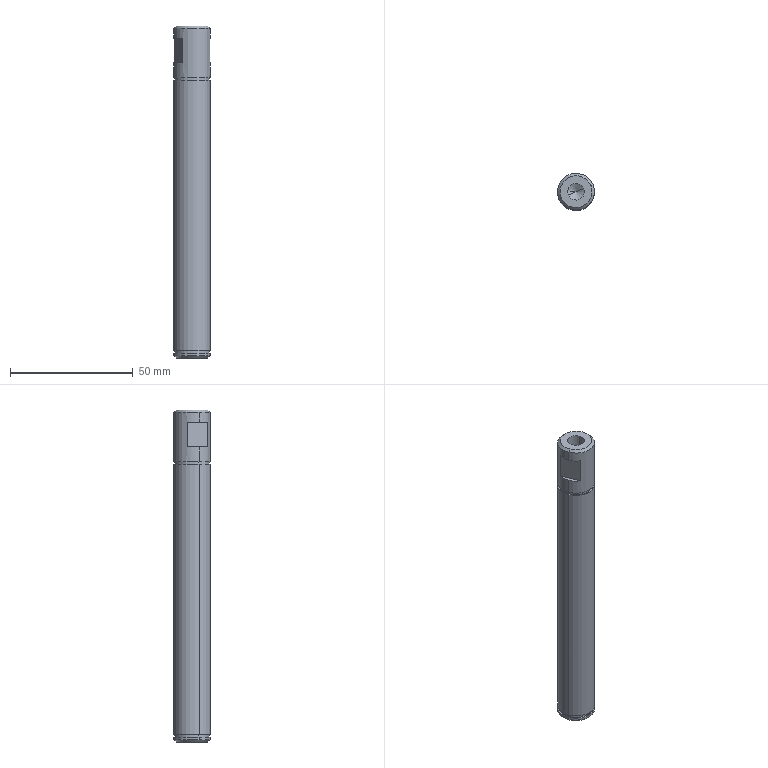Component | SolidWorks | TAR-01-28PaperSupportRollerAxis-1 | 1 solid | 30 faces | box 15 x 15 x 135.2 mm | volume 22680 mm3 | cylinder 12 | plane 12 | cone 6 | commonest cylinder face diameters 15 x6 14 x4 6.8 x2
build123d program:
from build123d import *

# Parameters (mm, degrees)
SKETCH1_R             = 7.5
BOSS_EXTRUDE1_DEPTH   = 5
BOSS_EXTRUDE2_DEPTH   = 10
SKETCH3_R             = 7.5
BOSS_EXTRUDE3_DEPTH   = 6
SKETCH4_R             = 7
BOSS_EXTRUDE4_DEPTH   = 1.1
SKETCH5_R             = 7.5
BOSS_EXTRUDE5_DEPTH   = 110
SKETCH6_R             = 7
BOSS_EXTRUDE6_DEPTH   = 1.1
SKETCH7_R             = 7.5
BOSS_EXTRUDE7_DEPTH   = 2
CHAMFER1_SIZE         = 1
M8_TAPPED_HOLE2_D     = 6.8
M8_TAPPED_HOLE2_DEPTH = 25
M8_TAPPED_HOLE2_TIP   = 2.043


with BuildPart() as part:
    # Sketch1 → Boss-Extrude1 (new body)
    with BuildSketch(Plane.XY):
        Circle(SKETCH1_R)
    extrude(amount=BOSS_EXTRUDE1_DEPTH)

    # Sketch2 → Boss-Extrude2 (add)
    with BuildSketch(Plane.XY.offset(5)):
        with BuildLine():
            Line((6, -4.5), (6, 4.5))
            ThreePointArc((6, 4.5), (0, 7.5), (-6, 4.5))
            Line((-6, 4.5), (-6, -4.5))
            ThreePointArc((-6, -4.5), (0, -7.5), (6, -4.5))
        make_face()
    extrude(amount=BOSS_EXTRUDE2_DEPTH)

    # Sketch3 → Boss-Extrude3 (add)
    with BuildSketch(Plane.XY.offset(15)):
        Circle(SKETCH3_R)
    extrude(amount=BOSS_EXTRUDE3_DEPTH)

    # Sketch4 → Boss-Extrude4 (add)
    with BuildSketch(Plane.XY.offset(21)):
        Circle(SKETCH4_R)
    extrude(amount=BOSS_EXTRUDE4_DEPTH)

    # Sketch5 → Boss-Extrude5 (add)
    with BuildSketch(Plane.XY.offset(22.1)):
        Circle(SKETCH5_R)
    extrude(amount=BOSS_EXTRUDE5_DEPTH)

    # Sketch6 → Boss-Extrude6 (add)
    with BuildSketch(Plane.XY.offset(132.1)):
        Circle(SKETCH6_R)
    extrude(amount=BOSS_EXTRUDE6_DEPTH)

    # Sketch7 → Boss-Extrude7 (add)
    with BuildSketch(Plane.XY.offset(133.2)):
        Circle(SKETCH7_R)
    extrude(amount=BOSS_EXTRUDE7_DEPTH)

    # Chamfer1
    chamfer1_edges = [part.edges().sort_by_distance(p)[0] for p in [
        (-7.5, 0, 0),
        (-7.5, 0, 135.2),
    ]]
    chamfer(chamfer1_edges, length=CHAMFER1_SIZE)

    # M8 Tapped Hole2
    with Locations(Plane(origin=(0, 0, 0), x_dir=(-1, 0, 0), z_dir=(0, 0, -1))):
        with Locations((0, 0)):
            Hole(M8_TAPPED_HOLE2_D / 2, depth=M8_TAPPED_HOLE2_DEPTH)
            with Locations((0, 0, -(M8_TAPPED_HOLE2_DEPTH + M8_TAPPED_HOLE2_TIP / 2))):  # 118° drill point
                Cone(0, M8_TAPPED_HOLE2_D / 2, M8_TAPPED_HOLE2_TIP, mode=Mode.SUBTRACT)


solid = part.part

# Placed as in the assembly
solid = solid.moved(Location((100.319, 9.938, -9.5), (-180, 0, -22.523)))
STEP:
#1=CARTESIAN_POINT('',(3.826,0.34,-1.358));
#2=VERTEX_POINT('',#1);
#3=CARTESIAN_POINT('',(4.073,0.4425,-1.358));
#4=VERTEX_POINT('',#3);
#5=CARTESIAN_POINT('',(3.95,0.3912,-1.358));
#6=DIRECTION('',(0.,0.,1.));
#7=DIRECTION('',(0.9237,0.383,0.));
#8=AXIS2_PLACEMENT_3D('',#5,#6,#7);
#9=CIRCLE('',#8,0.1339);
#10=EDGE_CURVE('',#2,#4,#9,.T.);
#11=ORIENTED_EDGE('',*,*,#10,.F.);
#12=CARTESIAN_POINT('',(3.826,0.34,-0.374));
#13=VERTEX_POINT('',#12);
#14=CARTESIAN_POINT('',(3.826,0.34,-0.374));
#15=DIRECTION('',(0.,0.,1.));
#16=VECTOR('',#15,39.37);
#17=LINE('',#14,#16);
#18=EDGE_CURVE('',#2,#13,#17,.T.);
#19=ORIENTED_EDGE('',*,*,#18,.T.);
#20=CARTESIAN_POINT('',(4.073,0.4425,-0.374));
#21=VERTEX_POINT('',#20);
#22=CARTESIAN_POINT('',(3.95,0.3912,-0.374));
#23=DIRECTION('',(0.,0.,1.));
#24=DIRECTION('',(0.9237,0.383,0.));
#25=AXIS2_PLACEMENT_3D('',#22,#23,#24);
#26=CIRCLE('',#25,0.1339);
#27=EDGE_CURVE('',#13,#21,#26,.T.);
#28=ORIENTED_EDGE('',*,*,#27,.T.);
#29=CARTESIAN_POINT('',(4.073,0.4425,-0.374));
#30=DIRECTION('',(0.,0.,1.));
#31=VECTOR('',#30,39.37);
#32=LINE('',#29,#31);
#33=EDGE_CURVE('',#4,#21,#32,.T.);
#34=ORIENTED_EDGE('',*,*,#33,.F.);
#35=EDGE_LOOP('',(#11,#19,#28,#34));
#36=FACE_OUTER_BOUND('',#35,.T.);
#37=CARTESIAN_POINT('',(3.95,0.3912,-0.374));
#38=DIRECTION('',(0.,0.,1.));
#39=DIRECTION('',(0.9237,0.383,0.));
#40=AXIS2_PLACEMENT_3D('',#37,#38,#39);
#41=CYLINDRICAL_SURFACE('',#40,0.1339);
#42=ADVANCED_FACE('',(#36),#41,.F.);
#43=CARTESIAN_POINT('',(3.95,0.3912,-1.439));
#44=VERTEX_POINT('',#43);
#45=CARTESIAN_POINT('',(4.073,0.4425,-1.358));
#46=DIRECTION('',(0.7918,0.3283,0.515));
#47=VECTOR('',#46,39.37);
#48=LINE('',#45,#47);
#49=EDGE_CURVE('',#44,#4,#48,.T.);
#50=ORIENTED_EDGE('',*,*,#49,.F.);
#51=CARTESIAN_POINT('',(3.826,0.34,-1.358));
#52=DIRECTION('',(-0.7918,-0.3283,0.515));
#53=VECTOR('',#52,39.37);
#54=LINE('',#51,#53);
#55=EDGE_CURVE('',#44,#2,#54,.T.);
#56=ORIENTED_EDGE('',*,*,#55,.T.);
#57=ORIENTED_EDGE('',*,*,#10,.T.);
#58=EDGE_LOOP('',(#50,#56,#57));
#59=FACE_OUTER_BOUND('',#58,.T.);
#60=CARTESIAN_POINT('',(3.95,0.3912,-1.358));
#61=DIRECTION('',(0.,0.,1.));
#62=DIRECTION('',(0.9237,0.383,0.));
#63=AXIS2_PLACEMENT_3D('',#60,#61,#62);
#64=CONICAL_SURFACE('',#63,0.1339,1.03);
#65=ADVANCED_FACE('',(#59),#64,.F.);
#66=CARTESIAN_POINT('',(3.713,0.2932,-5.697));
#67=VERTEX_POINT('',#66);
#68=CARTESIAN_POINT('',(4.186,0.4893,-5.697));
#69=VERTEX_POINT('',#68);
#70=CARTESIAN_POINT('',(3.95,0.3912,-5.697));
#71=DIRECTION('',(0.,0.,-1.));
#72=DIRECTION('',(-0.9237,-0.383,0.));
#73=AXIS2_PLACEMENT_3D('',#70,#71,#72);
#74=CIRCLE('',#73,0.2559);
#75=EDGE_CURVE('',#67,#69,#74,.T.);
#76=ORIENTED_EDGE('',*,*,#75,.F.);
#77=CARTESIAN_POINT('',(3.677,0.2781,-5.657));
#78=VERTEX_POINT('',#77);
#79=CARTESIAN_POINT('',(3.713,0.2932,-5.697));
#80=DIRECTION('',(-0.6532,-0.2709,0.7071));
#81=VECTOR('',#80,39.37);
#82=LINE('',#79,#81);
#83=EDGE_CURVE('',#67,#78,#82,.T.);
#84=ORIENTED_EDGE('',*,*,#83,.T.);
#85=CARTESIAN_POINT('',(4.222,0.5044,-5.657));
#86=VERTEX_POINT('',#85);
#87=CARTESIAN_POINT('',(3.95,0.3912,-5.657));
#88=DIRECTION('',(0.,0.,1.));
#89=DIRECTION('',(-0.9237,-0.383,0.));
#90=AXIS2_PLACEMENT_3D('',#87,#88,#89);
#91=CIRCLE('',#90,0.2953);
#92=EDGE_CURVE('',#86,#78,#91,.T.);
#93=ORIENTED_EDGE('',*,*,#92,.F.);
#94=CARTESIAN_POINT('',(4.186,0.4893,-5.697));
#95=DIRECTION('',(0.6532,0.2709,0.7071));
#96=VECTOR('',#95,39.37);
#97=LINE('',#94,#96);
#98=EDGE_CURVE('',#69,#86,#97,.T.);
#99=ORIENTED_EDGE('',*,*,#98,.F.);
#100=EDGE_LOOP('',(#76,#84,#93,#99));
#101=FACE_OUTER_BOUND('',#100,.T.);
#102=CARTESIAN_POINT('',(3.95,0.3912,-5.697));
#103=DIRECTION('',(0.,0.,1.));
#104=DIRECTION('',(0.9237,0.383,0.));
#105=AXIS2_PLACEMENT_3D('',#102,#103,#104);
#106=CONICAL_SURFACE('',#105,0.2559,0.7854);
#107=ADVANCED_FACE('',(#101),#106,.T.);
#108=CARTESIAN_POINT('',(4.186,0.4893,-0.374));
#109=VERTEX_POINT('',#108);
#110=CARTESIAN_POINT('',(3.713,0.2932,-0.374));
#111=VERTEX_POINT('',#110);
#112=CARTESIAN_POINT('',(3.95,0.3912,-0.374));
#113=DIRECTION('',(0.,0.,1.));
#114=DIRECTION('',(-0.9237,-0.383,0.));
#115=AXIS2_PLACEMENT_3D('',#112,#113,#114);
#116=CIRCLE('',#115,0.2559);
#117=EDGE_CURVE('',#109,#111,#116,.T.);
#118=ORIENTED_EDGE('',*,*,#117,.F.);
#119=CARTESIAN_POINT('',(4.222,0.5044,-0.4134));
#120=VERTEX_POINT('',#119);
#121=CARTESIAN_POINT('',(4.222,0.5044,-0.4134));
#122=DIRECTION('',(0.6532,0.2709,-0.7071));
#123=VECTOR('',#122,39.37);
#124=LINE('',#121,#123);
#125=EDGE_CURVE('',#109,#120,#124,.T.);
#126=ORIENTED_EDGE('',*,*,#125,.T.);
#127=CARTESIAN_POINT('',(3.677,0.2781,-0.4134));
#128=VERTEX_POINT('',#127);
#129=CARTESIAN_POINT('',(3.95,0.3912,-0.4134));
#130=DIRECTION('',(0.,0.,-1.));
#131=DIRECTION('',(-0.9237,-0.383,0.));
#132=AXIS2_PLACEMENT_3D('',#129,#130,#131);
#133=CIRCLE('',#132,0.2953);
#134=EDGE_CURVE('',#128,#120,#133,.T.);
#135=ORIENTED_EDGE('',*,*,#134,.F.);
#136=CARTESIAN_POINT('',(3.677,0.2781,-0.4134));
#137=DIRECTION('',(-0.6532,-0.2709,-0.7071));
#138=VECTOR('',#137,39.37);
#139=LINE('',#136,#138);
#140=EDGE_CURVE('',#111,#128,#139,.T.);
#141=ORIENTED_EDGE('',*,*,#140,.F.);
#142=EDGE_LOOP('',(#118,#126,#135,#141));
#143=FACE_OUTER_BOUND('',#142,.T.);
#144=CARTESIAN_POINT('',(3.95,0.3912,-0.4134));
#145=DIRECTION('',(0.,0.,-1.));
#146=DIRECTION('',(-0.9237,-0.383,0.));
#147=AXIS2_PLACEMENT_3D('',#144,#145,#146);
#148=CONICAL_SURFACE('',#147,0.2953,0.7854);
#149=ADVANCED_FACE('',(#143),#148,.T.);
#150=ORIENTED_EDGE('',*,*,#92,.T.);
#151=CARTESIAN_POINT('',(3.677,0.2781,-5.618));
#152=VERTEX_POINT('',#151);
#153=CARTESIAN_POINT('',(3.677,0.2781,-5.697));
#154=DIRECTION('',(0.,0.,1.));
#155=VECTOR('',#154,39.37);
#156=LINE('',#153,#155);
#157=EDGE_CURVE('',#78,#152,#156,.T.);
#158=ORIENTED_EDGE('',*,*,#157,.T.);
#159=CARTESIAN_POINT('',(4.222,0.5044,-5.618));
#160=VERTEX_POINT('',#159);
#161=CARTESIAN_POINT('',(3.95,0.3912,-5.618));
#162=DIRECTION('',(0.,0.,-1.));
#163=DIRECTION('',(-0.9237,-0.383,0.));
#164=AXIS2_PLACEMENT_3D('',#161,#162,#163);
#165=CIRCLE('',#164,0.2953);
#166=EDGE_CURVE('',#152,#160,#165,.T.);
#167=ORIENTED_EDGE('',*,*,#166,.T.);
#168=CARTESIAN_POINT('',(4.222,0.5044,-5.697));
#169=DIRECTION('',(0.,0.,1.));
#170=VECTOR('',#169,39.37);
#171=LINE('',#168,#170);
#172=EDGE_CURVE('',#86,#160,#171,.T.);
#173=ORIENTED_EDGE('',*,*,#172,.F.);
#174=EDGE_LOOP('',(#150,#158,#167,#173));
#175=FACE_OUTER_BOUND('',#174,.T.);
#176=CARTESIAN_POINT('',(3.95,0.3912,-5.697));
#177=DIRECTION('',(0.,0.,1.));
#178=DIRECTION('',(0.9237,0.383,0.));
#179=AXIS2_PLACEMENT_3D('',#176,#177,#178);
#180=CYLINDRICAL_SURFACE('',#179,0.2953);
#181=ADVANCED_FACE('',(#175),#180,.T.);
#182=CARTESIAN_POINT('',(3.695,0.2857,-5.618));
#183=VERTEX_POINT('',#182);
#184=CARTESIAN_POINT('',(4.204,0.4968,-5.618));
#185=VERTEX_POINT('',#184);
#186=CARTESIAN_POINT('',(3.95,0.3912,-5.618));
#187=DIRECTION('',(0.,0.,-1.));
#188=DIRECTION('',(-0.9237,-0.383,0.));
#189=AXIS2_PLACEMENT_3D('',#186,#187,#188);
#190=CIRCLE('',#189,0.2756);
#191=EDGE_CURVE('',#183,#185,#190,.T.);
#192=ORIENTED_EDGE('',*,*,#191,.F.);
#193=CARTESIAN_POINT('',(3.695,0.2857,-5.575));
#194=VERTEX_POINT('',#193);
#195=CARTESIAN_POINT('',(3.695,0.2857,-5.618));
#196=DIRECTION('',(0.,0.,1.));
#197=VECTOR('',#196,39.37);
#198=LINE('',#195,#197);
#199=EDGE_CURVE('',#183,#194,#198,.T.);
#200=ORIENTED_EDGE('',*,*,#199,.T.);
#201=CARTESIAN_POINT('',(4.204,0.4968,-5.575));
#202=VERTEX_POINT('',#201);
#203=CARTESIAN_POINT('',(3.95,0.3912,-5.575));
#204=DIRECTION('',(0.,0.,-1.));
#205=DIRECTION('',(-0.9237,-0.383,0.));
#206=AXIS2_PLACEMENT_3D('',#203,#204,#205);
#207=CIRCLE('',#206,0.2756);
#208=EDGE_CURVE('',#194,#202,#207,.T.);
#209=ORIENTED_EDGE('',*,*,#208,.T.);
#210=CARTESIAN_POINT('',(4.204,0.4968,-5.618));
#211=DIRECTION('',(0.,0.,1.));
#212=VECTOR('',#211,39.37);
#213=LINE('',#210,#212);
#214=EDGE_CURVE('',#185,#202,#213,.T.);
#215=ORIENTED_EDGE('',*,*,#214,.F.);
#216=EDGE_LOOP('',(#192,#200,#209,#215));
#217=FACE_OUTER_BOUND('',#216,.T.);
#218=CARTESIAN_POINT('',(3.95,0.3912,-5.618));
#219=DIRECTION('',(0.,0.,1.));
#220=DIRECTION('',(0.9237,0.383,0.));
#221=AXIS2_PLACEMENT_3D('',#218,#219,#220);
#222=CYLINDRICAL_SURFACE('',#221,0.2756);
#223=ADVANCED_FACE('',(#217),#222,.T.);
#224=CARTESIAN_POINT('',(3.677,0.2781,-5.575));
#225=VERTEX_POINT('',#224);
#226=CARTESIAN_POINT('',(4.222,0.5044,-5.575));
#227=VERTEX_POINT('',#226);
#228=CARTESIAN_POINT('',(3.95,0.3912,-5.575));
#229=DIRECTION('',(0.,0.,-1.));
#230=DIRECTION('',(-0.9237,-0.383,0.));
#231=AXIS2_PLACEMENT_3D('',#228,#229,#230);
#232=CIRCLE('',#231,0.2953);
#233=EDGE_CURVE('',#225,#227,#232,.T.);
#234=ORIENTED_EDGE('',*,*,#233,.F.);
#235=CARTESIAN_POINT('',(3.677,0.2781,-1.244));
#236=VERTEX_POINT('',#235);
#237=CARTESIAN_POINT('',(3.677,0.2781,-5.575));
#238=DIRECTION('',(0.,0.,1.));
#239=VECTOR('',#238,39.37);
#240=LINE('',#237,#239);
#241=EDGE_CURVE('',#225,#236,#240,.T.);
#242=ORIENTED_EDGE('',*,*,#241,.T.);
#243=CARTESIAN_POINT('',(4.222,0.5044,-1.244));
#244=VERTEX_POINT('',#243);
#245=CARTESIAN_POINT('',(3.95,0.3912,-1.244));
#246=DIRECTION('',(0.,0.,-1.));
#247=DIRECTION('',(-0.9237,-0.383,0.));
#248=AXIS2_PLACEMENT_3D('',#245,#246,#247);
#249=CIRCLE('',#248,0.2953);
#250=EDGE_CURVE('',#236,#244,#249,.T.);
#251=ORIENTED_EDGE('',*,*,#250,.T.);
#252=CARTESIAN_POINT('',(4.222,0.5044,-5.575));
#253=DIRECTION('',(0.,0.,1.));
#254=VECTOR('',#253,39.37);
#255=LINE('',#252,#254);
#256=EDGE_CURVE('',#227,#244,#255,.T.);
#257=ORIENTED_EDGE('',*,*,#256,.F.);
#258=EDGE_LOOP('',(#234,#242,#251,#257));
#259=FACE_OUTER_BOUND('',#258,.T.);
#260=CARTESIAN_POINT('',(3.95,0.3912,-5.575));
#261=DIRECTION('',(0.,0.,1.));
#262=DIRECTION('',(0.9237,0.383,0.));
#263=AXIS2_PLACEMENT_3D('',#260,#261,#262);
#264=CYLINDRICAL_SURFACE('',#263,0.2953);
#265=ADVANCED_FACE('',(#259),#264,.T.);
#266=CARTESIAN_POINT('',(3.695,0.2857,-1.244));
#267=VERTEX_POINT('',#266);
#268=CARTESIAN_POINT('',(4.204,0.4968,-1.244));
#269=VERTEX_POINT('',#268);
#270=CARTESIAN_POINT('',(3.95,0.3912,-1.244));
#271=DIRECTION('',(0.,0.,-1.));
#272=DIRECTION('',(-0.9237,-0.383,0.));
#273=AXIS2_PLACEMENT_3D('',#270,#271,#272);
#274=CIRCLE('',#273,0.2756);
#275=EDGE_CURVE('',#267,#269,#274,.T.);
#276=ORIENTED_EDGE('',*,*,#275,.F.);
#277=CARTESIAN_POINT('',(3.695,0.2857,-1.201));
#278=VERTEX_POINT('',#277);
#279=CARTESIAN_POINT('',(3.695,0.2857,-1.244));
#280=DIRECTION('',(0.,0.,1.));
#281=VECTOR('',#280,39.37);
#282=LINE('',#279,#281);
#283=EDGE_CURVE('',#267,#278,#282,.T.);
#284=ORIENTED_EDGE('',*,*,#283,.T.);
#285=CARTESIAN_POINT('',(4.204,0.4968,-1.201));
#286=VERTEX_POINT('',#285);
#287=CARTESIAN_POINT('',(3.95,0.3912,-1.201));
#288=DIRECTION('',(0.,0.,-1.));
#289=DIRECTION('',(-0.9237,-0.383,0.));
#290=AXIS2_PLACEMENT_3D('',#287,#288,#289);
#291=CIRCLE('',#290,0.2756);
#292=EDGE_CURVE('',#278,#286,#291,.T.);
#293=ORIENTED_EDGE('',*,*,#292,.T.);
#294=CARTESIAN_POINT('',(4.204,0.4968,-1.244));
#295=DIRECTION('',(0.,0.,1.));
#296=VECTOR('',#295,39.37);
#297=LINE('',#294,#296);
#298=EDGE_CURVE('',#269,#286,#297,.T.);
#299=ORIENTED_EDGE('',*,*,#298,.F.);
#300=EDGE_LOOP('',(#276,#284,#293,#299));
#301=FACE_OUTER_BOUND('',#300,.T.);
#302=CARTESIAN_POINT('',(3.95,0.3912,-1.244));
#303=DIRECTION('',(0.,0.,1.));
#304=DIRECTION('',(0.9237,0.383,0.));
#305=AXIS2_PLACEMENT_3D('',#302,#303,#304);
#306=CYLINDRICAL_SURFACE('',#305,0.2756);
#307=ADVANCED_FACE('',(#301),#306,.T.);
#308=CARTESIAN_POINT('',(3.677,0.2781,-1.201));
#309=VERTEX_POINT('',#308);
#310=CARTESIAN_POINT('',(4.222,0.5044,-1.201));
#311=VERTEX_POINT('',#310);
#312=CARTESIAN_POINT('',(3.95,0.3912,-1.201));
#313=DIRECTION('',(0.,0.,-1.));
#314=DIRECTION('',(-0.9237,-0.383,0.));
#315=AXIS2_PLACEMENT_3D('',#312,#313,#314);
#316=CIRCLE('',#315,0.2953);
#317=EDGE_CURVE('',#309,#311,#316,.T.);
#318=ORIENTED_EDGE('',*,*,#317,.F.);
#319=CARTESIAN_POINT('',(3.677,0.2781,-0.9646));
#320=VERTEX_POINT('',#319);
#321=CARTESIAN_POINT('',(3.677,0.2781,-0.5709));
#322=DIRECTION('',(0.,0.,1.));
#323=VECTOR('',#322,39.37);
#324=LINE('',#321,#323);
#325=EDGE_CURVE('',#309,#320,#324,.T.);
#326=ORIENTED_EDGE('',*,*,#325,.T.);
#327=CARTESIAN_POINT('',(3.664,0.4644,-0.9646));
#328=VERTEX_POINT('',#327);
#329=CARTESIAN_POINT('',(3.95,0.3912,-0.9646));
#330=DIRECTION('',(0.,0.,-1.));
#331=DIRECTION('',(-0.9237,-0.383,0.));
#332=AXIS2_PLACEMENT_3D('',#329,#330,#331);
#333=CIRCLE('',#332,0.2953);
#334=EDGE_CURVE('',#320,#328,#333,.T.);
#335=ORIENTED_EDGE('',*,*,#334,.T.);
#336=CARTESIAN_POINT('',(3.664,0.4644,-0.5709));
#337=VERTEX_POINT('',#336);
#338=CARTESIAN_POINT('',(3.664,0.4644,-0.9646));
#339=DIRECTION('',(0.,0.,1.));
#340=VECTOR('',#339,39.37);
#341=LINE('',#338,#340);
#342=EDGE_CURVE('',#328,#337,#341,.T.);
#343=ORIENTED_EDGE('',*,*,#342,.T.);
#344=CARTESIAN_POINT('',(3.677,0.2781,-0.5709));
#345=VERTEX_POINT('',#344);
#346=CARTESIAN_POINT('',(3.95,0.3912,-0.5709));
#347=DIRECTION('',(0.,0.,-1.));
#348=DIRECTION('',(-0.9237,-0.383,0.));
#349=AXIS2_PLACEMENT_3D('',#346,#347,#348);
#350=CIRCLE('',#349,0.2953);
#351=EDGE_CURVE('',#345,#337,#350,.T.);
#352=ORIENTED_EDGE('',*,*,#351,.F.);
#353=CARTESIAN_POINT('',(3.677,0.2781,-0.5709));
#354=DIRECTION('',(0.,0.,1.));
#355=VECTOR('',#354,39.37);
#356=LINE('',#353,#355);
#357=EDGE_CURVE('',#345,#128,#356,.T.);
#358=ORIENTED_EDGE('',*,*,#357,.T.);
#359=ORIENTED_EDGE('',*,*,#134,.T.);
#360=CARTESIAN_POINT('',(4.222,0.5044,-0.5709));
#361=VERTEX_POINT('',#360);
#362=CARTESIAN_POINT('',(4.222,0.5044,-0.5709));
#363=DIRECTION('',(0.,0.,1.));
#364=VECTOR('',#363,39.37);
#365=LINE('',#362,#364);
#366=EDGE_CURVE('',#361,#120,#365,.T.);
#367=ORIENTED_EDGE('',*,*,#366,.F.);
#368=CARTESIAN_POINT('',(4.1,0.6454,-0.5709));
#369=VERTEX_POINT('',#368);
#370=CARTESIAN_POINT('',(3.95,0.3912,-0.5709));
#371=DIRECTION('',(0.,0.,-1.));
#372=DIRECTION('',(-0.9237,-0.383,0.));
#373=AXIS2_PLACEMENT_3D('',#370,#371,#372);
#374=CIRCLE('',#373,0.2953);
#375=EDGE_CURVE('',#369,#361,#374,.T.);
#376=ORIENTED_EDGE('',*,*,#375,.F.);
#377=CARTESIAN_POINT('',(4.1,0.6454,-0.9646));
#378=VERTEX_POINT('',#377);
#379=CARTESIAN_POINT('',(4.1,0.6454,-0.9646));
#380=DIRECTION('',(0.,0.,1.));
#381=VECTOR('',#380,39.37);
#382=LINE('',#379,#381);
#383=EDGE_CURVE('',#378,#369,#382,.T.);
#384=ORIENTED_EDGE('',*,*,#383,.F.);
#385=CARTESIAN_POINT('',(4.222,0.5044,-0.9646));
#386=VERTEX_POINT('',#385);
#387=CARTESIAN_POINT('',(3.95,0.3912,-0.9646));
#388=DIRECTION('',(0.,0.,-1.));
#389=DIRECTION('',(-0.9237,-0.383,0.));
#390=AXIS2_PLACEMENT_3D('',#387,#388,#389);
#391=CIRCLE('',#390,0.2953);
#392=EDGE_CURVE('',#378,#386,#391,.T.);
#393=ORIENTED_EDGE('',*,*,#392,.T.);
#394=CARTESIAN_POINT('',(4.222,0.5044,-0.5709));
#395=DIRECTION('',(0.,0.,1.));
#396=VECTOR('',#395,39.37);
#397=LINE('',#394,#396);
#398=EDGE_CURVE('',#311,#386,#397,.T.);
#399=ORIENTED_EDGE('',*,*,#398,.F.);
#400=EDGE_LOOP('',(#318,#326,#335,#343,#352,#358,#359,#367,#376,#384,#393,#399));
#401=FACE_OUTER_BOUND('',#400,.T.);
#402=CARTESIAN_POINT('',(3.95,0.3912,-0.5709));
#403=DIRECTION('',(0.,0.,1.));
#404=DIRECTION('',(0.9237,0.383,0.));
#405=AXIS2_PLACEMENT_3D('',#402,#403,#404);
#406=CYLINDRICAL_SURFACE('',#405,0.2953);
#407=ADVANCED_FACE('',(#401),#406,.T.);
#408=CARTESIAN_POINT('',(4.236,0.3181,-0.5709));
#409=VERTEX_POINT('',#408);
#410=CARTESIAN_POINT('',(4.236,0.3181,-0.5709));
#411=DIRECTION('',(0.383,-0.9237,0.));
#412=VECTOR('',#411,39.37);
#413=LINE('',#410,#412);
#414=EDGE_CURVE('',#369,#409,#413,.T.);
#415=ORIENTED_EDGE('',*,*,#414,.F.);
#416=ORIENTED_EDGE('',*,*,#375,.T.);
#417=CARTESIAN_POINT('',(3.95,0.3912,-0.5709));
#418=DIRECTION('',(0.,0.,-1.));
#419=DIRECTION('',(-0.9237,-0.383,0.));
#420=AXIS2_PLACEMENT_3D('',#417,#418,#419);
#421=CIRCLE('',#420,0.2953);
#422=EDGE_CURVE('',#361,#409,#421,.T.);
#423=ORIENTED_EDGE('',*,*,#422,.T.);
#424=EDGE_LOOP('',(#415,#416,#423));
#425=FACE_OUTER_BOUND('',#424,.T.);
#426=CARTESIAN_POINT('',(3.95,0.3912,-0.5709));
#427=DIRECTION('',(0.,0.,-1.));
#428=DIRECTION('',(-0.9237,-0.383,0.));
#429=AXIS2_PLACEMENT_3D('',#426,#427,#428);
#430=PLANE('',#429);
#431=ADVANCED_FACE('',(#425),#430,.T.);
#432=ORIENTED_EDGE('',*,*,#325,.F.);
#433=CARTESIAN_POINT('',(3.95,0.3912,-1.201));
#434=DIRECTION('',(0.,0.,-1.));
#435=DIRECTION('',(-0.9237,-0.383,0.));
#436=AXIS2_PLACEMENT_3D('',#433,#434,#435);
#437=CIRCLE('',#436,0.2953);
#438=EDGE_CURVE('',#311,#309,#437,.T.);
#439=ORIENTED_EDGE('',*,*,#438,.F.);
#440=ORIENTED_EDGE('',*,*,#398,.T.);
#441=CARTESIAN_POINT('',(4.236,0.3181,-0.9646));
#442=VERTEX_POINT('',#441);
#443=CARTESIAN_POINT('',(3.95,0.3912,-0.9646));
#444=DIRECTION('',(0.,0.,-1.));
#445=DIRECTION('',(-0.9237,-0.383,0.));
#446=AXIS2_PLACEMENT_3D('',#443,#444,#445);
#447=CIRCLE('',#446,0.2953);
#448=EDGE_CURVE('',#386,#442,#447,.T.);
#449=ORIENTED_EDGE('',*,*,#448,.T.);
#450=CARTESIAN_POINT('',(4.236,0.3181,-0.9646));
#451=DIRECTION('',(0.,0.,1.));
#452=VECTOR('',#451,39.37);
#453=LINE('',#450,#452);
#454=EDGE_CURVE('',#442,#409,#453,.T.);
#455=ORIENTED_EDGE('',*,*,#454,.T.);
#456=ORIENTED_EDGE('',*,*,#422,.F.);
#457=ORIENTED_EDGE('',*,*,#366,.T.);
#458=CARTESIAN_POINT('',(3.95,0.3912,-0.4134));
#459=DIRECTION('',(0.,0.,-1.));
#460=DIRECTION('',(-0.9237,-0.383,0.));
#461=AXIS2_PLACEMENT_3D('',#458,#459,#460);
#462=CIRCLE('',#461,0.2953);
#463=EDGE_CURVE('',#120,#128,#462,.T.);
#464=ORIENTED_EDGE('',*,*,#463,.T.);
#465=ORIENTED_EDGE('',*,*,#357,.F.);
#466=CARTESIAN_POINT('',(3.799,0.1371,-0.5709));
#467=VERTEX_POINT('',#466);
#468=CARTESIAN_POINT('',(3.95,0.3912,-0.5709));
#469=DIRECTION('',(0.,0.,-1.));
#470=DIRECTION('',(-0.9237,-0.383,0.));
#471=AXIS2_PLACEMENT_3D('',#468,#469,#470);
#472=CIRCLE('',#471,0.2953);
#473=EDGE_CURVE('',#467,#345,#472,.T.);
#474=ORIENTED_EDGE('',*,*,#473,.F.);
#475=CARTESIAN_POINT('',(3.799,0.1371,-0.9646));
#476=VERTEX_POINT('',#475);
#477=CARTESIAN_POINT('',(3.799,0.1371,-0.9646));
#478=DIRECTION('',(0.,0.,1.));
#479=VECTOR('',#478,39.37);
#480=LINE('',#477,#479);
#481=EDGE_CURVE('',#476,#467,#480,.T.);
#482=ORIENTED_EDGE('',*,*,#481,.F.);
#483=CARTESIAN_POINT('',(3.95,0.3912,-0.9646));
#484=DIRECTION('',(0.,0.,-1.));
#485=DIRECTION('',(-0.9237,-0.383,0.));
#486=AXIS2_PLACEMENT_3D('',#483,#484,#485);
#487=CIRCLE('',#486,0.2953);
#488=EDGE_CURVE('',#476,#320,#487,.T.);
#489=ORIENTED_EDGE('',*,*,#488,.T.);
#490=EDGE_LOOP('',(#432,#439,#440,#449,#455,#456,#457,#464,#465,#474,#482,#489));
#491=FACE_OUTER_BOUND('',#490,.T.);
#492=CARTESIAN_POINT('',(3.95,0.3912,-0.5709));
#493=DIRECTION('',(0.,0.,1.));
#494=DIRECTION('',(0.9237,0.383,0.));
#495=AXIS2_PLACEMENT_3D('',#492,#493,#494);
#496=CYLINDRICAL_SURFACE('',#495,0.2953);
#497=ADVANCED_FACE('',(#491),#496,.T.);
#498=CARTESIAN_POINT('',(3.799,0.1371,-0.5709));
#499=DIRECTION('',(-0.383,0.9237,0.));
#500=VECTOR('',#499,39.37);
#501=LINE('',#498,#500);
#502=EDGE_CURVE('',#467,#337,#501,.T.);
#503=ORIENTED_EDGE('',*,*,#502,.F.);
#504=ORIENTED_EDGE('',*,*,#473,.T.);
#505=ORIENTED_EDGE('',*,*,#351,.T.);
#506=EDGE_LOOP('',(#503,#504,#505));
#507=FACE_OUTER_BOUND('',#506,.T.);
#508=CARTESIAN_POINT('',(3.95,0.3912,-0.5709));
#509=DIRECTION('',(0.,0.,-1.));
#510=DIRECTION('',(-0.9237,-0.383,0.));
#511=AXIS2_PLACEMENT_3D('',#508,#509,#510);
#512=PLANE('',#511);
#513=ADVANCED_FACE('',(#507),#512,.T.);
#514=CARTESIAN_POINT('',(3.95,0.3912,-0.374));
#515=DIRECTION('',(0.,0.,1.));
#516=DIRECTION('',(0.9237,0.383,0.));
#517=AXIS2_PLACEMENT_3D('',#514,#515,#516);
#518=CIRCLE('',#517,0.1339);
#519=EDGE_CURVE('',#21,#13,#518,.T.);
#520=ORIENTED_EDGE('',*,*,#519,.F.);
#521=ORIENTED_EDGE('',*,*,#27,.F.);
#522=EDGE_LOOP('',(#520,#521));
#523=FACE_BOUND('',#522,.T.);
#524=CARTESIAN_POINT('',(3.95,0.3912,-0.374));
#525=DIRECTION('',(0.,0.,1.));
#526=DIRECTION('',(-0.9237,-0.383,0.));
#527=AXIS2_PLACEMENT_3D('',#524,#525,#526);
#528=CIRCLE('',#527,0.2559);
#529=EDGE_CURVE('',#111,#109,#528,.T.);
#530=ORIENTED_EDGE('',*,*,#529,.T.);
#531=ORIENTED_EDGE('',*,*,#117,.T.);
#532=EDGE_LOOP('',(#530,#531));
#533=FACE_OUTER_BOUND('',#532,.T.);
#534=CARTESIAN_POINT('',(3.95,0.3912,-0.374));
#535=DIRECTION('',(0.,0.,-1.));
#536=DIRECTION('',(-0.9237,-0.383,0.));
#537=AXIS2_PLACEMENT_3D('',#534,#535,#536);
#538=PLANE('',#537);
#539=ADVANCED_FACE('',(#523,#533),#538,.F.);
#540=ORIENTED_EDGE('',*,*,#502,.T.);
#541=ORIENTED_EDGE('',*,*,#342,.F.);
#542=CARTESIAN_POINT('',(3.799,0.1371,-0.9646));
#543=DIRECTION('',(-0.383,0.9237,0.));
#544=VECTOR('',#543,39.37);
#545=LINE('',#542,#544);
#546=EDGE_CURVE('',#476,#328,#545,.T.);
#547=ORIENTED_EDGE('',*,*,#546,.F.);
#548=ORIENTED_EDGE('',*,*,#481,.T.);
#549=EDGE_LOOP('',(#540,#541,#547,#548));
#550=FACE_OUTER_BOUND('',#549,.T.);
#551=CARTESIAN_POINT('',(3.799,0.1371,-0.9646));
#552=DIRECTION('',(0.9237,0.383,0.));
#553=DIRECTION('',(0.,0.,-1.));
#554=AXIS2_PLACEMENT_3D('',#551,#552,#553);
#555=PLANE('',#554);
#556=ADVANCED_FACE('',(#550),#555,.F.);
#557=ORIENTED_EDGE('',*,*,#414,.T.);
#558=ORIENTED_EDGE('',*,*,#454,.F.);
#559=CARTESIAN_POINT('',(4.236,0.3181,-0.9646));
#560=DIRECTION('',(0.383,-0.9237,0.));
#561=VECTOR('',#560,39.37);
#562=LINE('',#559,#561);
#563=EDGE_CURVE('',#378,#442,#562,.T.);
#564=ORIENTED_EDGE('',*,*,#563,.F.);
#565=ORIENTED_EDGE('',*,*,#383,.T.);
#566=EDGE_LOOP('',(#557,#558,#564,#565));
#567=FACE_OUTER_BOUND('',#566,.T.);
#568=CARTESIAN_POINT('',(4.236,0.3181,-0.9646));
#569=DIRECTION('',(-0.9237,-0.383,0.));
#570=DIRECTION('',(0.,0.,1.));
#571=AXIS2_PLACEMENT_3D('',#568,#569,#570);
#572=PLANE('',#571);
#573=ADVANCED_FACE('',(#567),#572,.F.);
#574=ORIENTED_EDGE('',*,*,#488,.F.);
#575=ORIENTED_EDGE('',*,*,#546,.T.);
#576=ORIENTED_EDGE('',*,*,#334,.F.);
#577=EDGE_LOOP('',(#574,#575,#576));
#578=FACE_OUTER_BOUND('',#577,.T.);
#579=CARTESIAN_POINT('',(3.95,0.3912,-0.9646));
#580=DIRECTION('',(0.,0.,-1.));
#581=DIRECTION('',(-0.9237,-0.383,0.));
#582=AXIS2_PLACEMENT_3D('',#579,#580,#581);
#583=PLANE('',#582);
#584=ADVANCED_FACE('',(#578),#583,.F.);
#585=ORIENTED_EDGE('',*,*,#392,.F.);
#586=ORIENTED_EDGE('',*,*,#563,.T.);
#587=ORIENTED_EDGE('',*,*,#448,.F.);
#588=EDGE_LOOP('',(#585,#586,#587));
#589=FACE_OUTER_BOUND('',#588,.T.);
#590=CARTESIAN_POINT('',(3.95,0.3912,-0.9646));
#591=DIRECTION('',(0.,0.,-1.));
#592=DIRECTION('',(-0.9237,-0.383,0.));
#593=AXIS2_PLACEMENT_3D('',#590,#591,#592);
#594=PLANE('',#593);
#595=ADVANCED_FACE('',(#589),#594,.F.);
#596=CARTESIAN_POINT('',(3.95,0.3912,-1.201));
#597=DIRECTION('',(0.,0.,-1.));
#598=DIRECTION('',(-0.9237,-0.383,0.));
#599=AXIS2_PLACEMENT_3D('',#596,#597,#598);
#600=CIRCLE('',#599,0.2756);
#601=EDGE_CURVE('',#286,#278,#600,.T.);
#602=ORIENTED_EDGE('',*,*,#601,.F.);
#603=ORIENTED_EDGE('',*,*,#292,.F.);
#604=EDGE_LOOP('',(#602,#603));
#605=FACE_BOUND('',#604,.T.);
#606=ORIENTED_EDGE('',*,*,#438,.T.);
#607=ORIENTED_EDGE('',*,*,#317,.T.);
#608=EDGE_LOOP('',(#606,#607));
#609=FACE_OUTER_BOUND('',#608,.T.);
#610=CARTESIAN_POINT('',(3.95,0.3912,-1.201));
#611=DIRECTION('',(0.,0.,-1.));
#612=DIRECTION('',(-0.9237,-0.383,0.));
#613=AXIS2_PLACEMENT_3D('',#610,#611,#612);
#614=PLANE('',#613);
#615=ADVANCED_FACE('',(#605,#609),#614,.T.);
#616=ORIENTED_EDGE('',*,*,#283,.F.);
#617=CARTESIAN_POINT('',(3.95,0.3912,-1.244));
#618=DIRECTION('',(0.,0.,-1.));
#619=DIRECTION('',(-0.9237,-0.383,0.));
#620=AXIS2_PLACEMENT_3D('',#617,#618,#619);
#621=CIRCLE('',#620,0.2756);
#622=EDGE_CURVE('',#269,#267,#621,.T.);
#623=ORIENTED_EDGE('',*,*,#622,.F.);
#624=ORIENTED_EDGE('',*,*,#298,.T.);
#625=ORIENTED_EDGE('',*,*,#601,.T.);
#626=EDGE_LOOP('',(#616,#623,#624,#625));
#627=FACE_OUTER_BOUND('',#626,.T.);
#628=CARTESIAN_POINT('',(3.95,0.3912,-1.244));
#629=DIRECTION('',(0.,0.,1.));
#630=DIRECTION('',(0.9237,0.383,0.));
#631=AXIS2_PLACEMENT_3D('',#628,#629,#630);
#632=CYLINDRICAL_SURFACE('',#631,0.2756);
#633=ADVANCED_FACE('',(#627),#632,.T.);
#634=ORIENTED_EDGE('',*,*,#241,.F.);
#635=CARTESIAN_POINT('',(3.95,0.3912,-5.575));
#636=DIRECTION('',(0.,0.,-1.));
#637=DIRECTION('',(-0.9237,-0.383,0.));
#638=AXIS2_PLACEMENT_3D('',#635,#636,#637);
#639=CIRCLE('',#638,0.2953);
#640=EDGE_CURVE('',#227,#225,#639,.T.);
#641=ORIENTED_EDGE('',*,*,#640,.F.);
#642=ORIENTED_EDGE('',*,*,#256,.T.);
#643=CARTESIAN_POINT('',(3.95,0.3912,-1.244));
#644=DIRECTION('',(0.,0.,-1.));
#645=DIRECTION('',(-0.9237,-0.383,0.));
#646=AXIS2_PLACEMENT_3D('',#643,#644,#645);
#647=CIRCLE('',#646,0.2953);
#648=EDGE_CURVE('',#244,#236,#647,.T.);
#649=ORIENTED_EDGE('',*,*,#648,.T.);
#650=EDGE_LOOP('',(#634,#641,#642,#649));
#651=FACE_OUTER_BOUND('',#650,.T.);
#652=CARTESIAN_POINT('',(3.95,0.3912,-5.575));
#653=DIRECTION('',(0.,0.,1.));
#654=DIRECTION('',(0.9237,0.383,0.));
#655=AXIS2_PLACEMENT_3D('',#652,#653,#654);
#656=CYLINDRICAL_SURFACE('',#655,0.2953);
#657=ADVANCED_FACE('',(#651),#656,.T.);
#658=CARTESIAN_POINT('',(3.95,0.3912,-5.575));
#659=DIRECTION('',(0.,0.,-1.));
#660=DIRECTION('',(-0.9237,-0.383,0.));
#661=AXIS2_PLACEMENT_3D('',#658,#659,#660);
#662=CIRCLE('',#661,0.2756);
#663=EDGE_CURVE('',#202,#194,#662,.T.);
#664=ORIENTED_EDGE('',*,*,#663,.F.);
#665=ORIENTED_EDGE('',*,*,#208,.F.);
#666=EDGE_LOOP('',(#664,#665));
#667=FACE_BOUND('',#666,.T.);
#668=ORIENTED_EDGE('',*,*,#640,.T.);
#669=ORIENTED_EDGE('',*,*,#233,.T.);
#670=EDGE_LOOP('',(#668,#669));
#671=FACE_OUTER_BOUND('',#670,.T.);
#672=CARTESIAN_POINT('',(3.95,0.3912,-5.575));
#673=DIRECTION('',(0.,0.,-1.));
#674=DIRECTION('',(-0.9237,-0.383,0.));
#675=AXIS2_PLACEMENT_3D('',#672,#673,#674);
#676=PLANE('',#675);
#677=ADVANCED_FACE('',(#667,#671),#676,.T.);
#678=ORIENTED_EDGE('',*,*,#622,.T.);
#679=ORIENTED_EDGE('',*,*,#275,.T.);
#680=EDGE_LOOP('',(#678,#679));
#681=FACE_BOUND('',#680,.T.);
#682=ORIENTED_EDGE('',*,*,#648,.F.);
#683=ORIENTED_EDGE('',*,*,#250,.F.);
#684=EDGE_LOOP('',(#682,#683));
#685=FACE_OUTER_BOUND('',#684,.T.);
#686=CARTESIAN_POINT('',(3.95,0.3912,-1.244));
#687=DIRECTION('',(0.,0.,-1.));
#688=DIRECTION('',(-0.9237,-0.383,0.));
#689=AXIS2_PLACEMENT_3D('',#686,#687,#688);
#690=PLANE('',#689);
#691=ADVANCED_FACE('',(#681,#685),#690,.F.);
#692=ORIENTED_EDGE('',*,*,#199,.F.);
#693=CARTESIAN_POINT('',(3.95,0.3912,-5.618));
#694=DIRECTION('',(0.,0.,-1.));
#695=DIRECTION('',(-0.9237,-0.383,0.));
#696=AXIS2_PLACEMENT_3D('',#693,#694,#695);
#697=CIRCLE('',#696,0.2756);
#698=EDGE_CURVE('',#185,#183,#697,.T.);
#699=ORIENTED_EDGE('',*,*,#698,.F.);
#700=ORIENTED_EDGE('',*,*,#214,.T.);
#701=ORIENTED_EDGE('',*,*,#663,.T.);
#702=EDGE_LOOP('',(#692,#699,#700,#701));
#703=FACE_OUTER_BOUND('',#702,.T.);
#704=CARTESIAN_POINT('',(3.95,0.3912,-5.618));
#705=DIRECTION('',(0.,0.,1.));
#706=DIRECTION('',(0.9237,0.383,0.));
#707=AXIS2_PLACEMENT_3D('',#704,#705,#706);
#708=CYLINDRICAL_SURFACE('',#707,0.2756);
#709=ADVANCED_FACE('',(#703),#708,.T.);
#710=ORIENTED_EDGE('',*,*,#157,.F.);
#711=CARTESIAN_POINT('',(3.95,0.3912,-5.657));
#712=DIRECTION('',(0.,0.,1.));
#713=DIRECTION('',(-0.9237,-0.383,0.));
#714=AXIS2_PLACEMENT_3D('',#711,#712,#713);
#715=CIRCLE('',#714,0.2953);
#716=EDGE_CURVE('',#78,#86,#715,.T.);
#717=ORIENTED_EDGE('',*,*,#716,.T.);
#718=ORIENTED_EDGE('',*,*,#172,.T.);
#719=CARTESIAN_POINT('',(3.95,0.3912,-5.618));
#720=DIRECTION('',(0.,0.,-1.));
#721=DIRECTION('',(-0.9237,-0.383,0.));
#722=AXIS2_PLACEMENT_3D('',#719,#720,#721);
#723=CIRCLE('',#722,0.2953);
#724=EDGE_CURVE('',#160,#152,#723,.T.);
#725=ORIENTED_EDGE('',*,*,#724,.T.);
#726=EDGE_LOOP('',(#710,#717,#718,#725));
#727=FACE_OUTER_BOUND('',#726,.T.);
#728=CARTESIAN_POINT('',(3.95,0.3912,-5.697));
#729=DIRECTION('',(0.,0.,1.));
#730=DIRECTION('',(0.9237,0.383,0.));
#731=AXIS2_PLACEMENT_3D('',#728,#729,#730);
#732=CYLINDRICAL_SURFACE('',#731,0.2953);
#733=ADVANCED_FACE('',(#727),#732,.T.);
#734=CARTESIAN_POINT('',(3.95,0.3912,-5.697));
#735=DIRECTION('',(0.,0.,-1.));
#736=DIRECTION('',(-0.9237,-0.383,0.));
#737=AXIS2_PLACEMENT_3D('',#734,#735,#736);
#738=CIRCLE('',#737,0.2559);
#739=EDGE_CURVE('',#69,#67,#738,.T.);
#740=ORIENTED_EDGE('',*,*,#739,.T.);
#741=ORIENTED_EDGE('',*,*,#75,.T.);
#742=EDGE_LOOP('',(#740,#741));
#743=FACE_OUTER_BOUND('',#742,.T.);
#744=CARTESIAN_POINT('',(3.95,0.3912,-5.697));
#745=DIRECTION('',(0.,0.,-1.));
#746=DIRECTION('',(-0.9237,-0.383,0.));
#747=AXIS2_PLACEMENT_3D('',#744,#745,#746);
#748=PLANE('',#747);
#749=ADVANCED_FACE('',(#743),#748,.T.);
#750=ORIENTED_EDGE('',*,*,#698,.T.);
#751=ORIENTED_EDGE('',*,*,#191,.T.);
#752=EDGE_LOOP('',(#750,#751));
#753=FACE_BOUND('',#752,.T.);
#754=ORIENTED_EDGE('',*,*,#724,.F.);
#755=ORIENTED_EDGE('',*,*,#166,.F.);
#756=EDGE_LOOP('',(#754,#755));
#757=FACE_OUTER_BOUND('',#756,.T.);
#758=CARTESIAN_POINT('',(3.95,0.3912,-5.618));
#759=DIRECTION('',(0.,0.,-1.));
#760=DIRECTION('',(-0.9237,-0.383,0.));
#761=AXIS2_PLACEMENT_3D('',#758,#759,#760);
#762=PLANE('',#761);
#763=ADVANCED_FACE('',(#753,#757),#762,.F.);
#764=ORIENTED_EDGE('',*,*,#125,.F.);
#765=ORIENTED_EDGE('',*,*,#529,.F.);
#766=ORIENTED_EDGE('',*,*,#140,.T.);
#767=ORIENTED_EDGE('',*,*,#463,.F.);
#768=EDGE_LOOP('',(#764,#765,#766,#767));
#769=FACE_OUTER_BOUND('',#768,.T.);
#770=CARTESIAN_POINT('',(3.95,0.3912,-0.4134));
#771=DIRECTION('',(0.,0.,-1.));
#772=DIRECTION('',(-0.9237,-0.383,0.));
#773=AXIS2_PLACEMENT_3D('',#770,#771,#772);
#774=CONICAL_SURFACE('',#773,0.2953,0.7854);
#775=ADVANCED_FACE('',(#769),#774,.T.);
#776=ORIENTED_EDGE('',*,*,#83,.F.);
#777=ORIENTED_EDGE('',*,*,#739,.F.);
#778=ORIENTED_EDGE('',*,*,#98,.T.);
#779=ORIENTED_EDGE('',*,*,#716,.F.);
#780=EDGE_LOOP('',(#776,#777,#778,#779));
#781=FACE_OUTER_BOUND('',#780,.T.);
#782=CARTESIAN_POINT('',(3.95,0.3912,-5.697));
#783=DIRECTION('',(0.,0.,1.));
#784=DIRECTION('',(0.9237,0.383,0.));
#785=AXIS2_PLACEMENT_3D('',#782,#783,#784);
#786=CONICAL_SURFACE('',#785,0.2559,0.7854);
#787=ADVANCED_FACE('',(#781),#786,.T.);
#788=ORIENTED_EDGE('',*,*,#55,.F.);
#789=ORIENTED_EDGE('',*,*,#49,.T.);
#790=CARTESIAN_POINT('',(3.95,0.3912,-1.358));
#791=DIRECTION('',(0.,0.,1.));
#792=DIRECTION('',(0.9237,0.383,0.));
#793=AXIS2_PLACEMENT_3D('',#790,#791,#792);
#794=CIRCLE('',#793,0.1339);
#795=EDGE_CURVE('',#4,#2,#794,.T.);
#796=ORIENTED_EDGE('',*,*,#795,.T.);
#797=EDGE_LOOP('',(#788,#789,#796));
#798=FACE_OUTER_BOUND('',#797,.T.);
#799=CARTESIAN_POINT('',(3.95,0.3912,-1.358));
#800=DIRECTION('',(0.,0.,1.));
#801=DIRECTION('',(0.9237,0.383,0.));
#802=AXIS2_PLACEMENT_3D('',#799,#800,#801);
#803=CONICAL_SURFACE('',#802,0.1339,1.03);
#804=ADVANCED_FACE('',(#798),#803,.F.);
#805=ORIENTED_EDGE('',*,*,#18,.F.);
#806=ORIENTED_EDGE('',*,*,#795,.F.);
#807=ORIENTED_EDGE('',*,*,#33,.T.);
#808=ORIENTED_EDGE('',*,*,#519,.T.);
#809=EDGE_LOOP('',(#805,#806,#807,#808));
#810=FACE_OUTER_BOUND('',#809,.T.);
#811=CARTESIAN_POINT('',(3.95,0.3912,-0.374));
#812=DIRECTION('',(0.,0.,1.));
#813=DIRECTION('',(0.9237,0.383,0.));
#814=AXIS2_PLACEMENT_3D('',#811,#812,#813);
#815=CYLINDRICAL_SURFACE('',#814,0.1339);
#816=ADVANCED_FACE('',(#810),#815,.F.);
#817=CLOSED_SHELL('',(#42,#65,#107,#149,#181,#223,#265,#307,#407,#431,#497,#513,#539,#556,#573,#584,#595,#615,#633,#657,#677,#691,#709,#733,#749,#763,#775,#787,#804,#816));
#818=MANIFOLD_SOLID_BREP('',#817);
#819=CARTESIAN_POINT('',(0.,0.,0.));
#820=DIRECTION('',(0.,0.,1.));
#821=DIRECTION('',(1.,0.,0.));
#822=AXIS2_PLACEMENT_3D('',#819,#820,#821);
#823=(LENGTH_UNIT()NAMED_UNIT(*)SI_UNIT($,.METRE.));
#824=LENGTH_MEASURE_WITH_UNIT(LENGTH_MEASURE(0.0254),#823);
#825=DIMENSIONAL_EXPONENTS(1.,0.,0.,0.,0.,0.,0.);
#826=(CONVERSION_BASED_UNIT('',#824)LENGTH_UNIT()NAMED_UNIT(#825));
#827=UNCERTAINTY_MEASURE_WITH_UNIT(LENGTH_MEASURE(0.00001),#826,'','');
#828=(NAMED_UNIT(*)PLANE_ANGLE_UNIT()SI_UNIT($,.RADIAN.));
#829=(NAMED_UNIT(*)SI_UNIT($,.STERADIAN.)SOLID_ANGLE_UNIT());
#830=(GEOMETRIC_REPRESENTATION_CONTEXT(3)GLOBAL_UNCERTAINTY_ASSIGNED_CONTEXT((#827))GLOBAL_UNIT_ASSIGNED_CONTEXT((#826,#828,#829))REPRESENTATION_CONTEXT('',''));
#831=ADVANCED_BREP_SHAPE_REPRESENTATION('',(#818,#822),#830);
#832=COLOUR_RGB('',0.7922,0.8196,0.9333);
#833=FILL_AREA_STYLE_COLOUR('',#832);
#834=FILL_AREA_STYLE('',(#833));
#835=SURFACE_STYLE_FILL_AREA(#834);
#836=SURFACE_SIDE_STYLE('',(#835));
#837=SURFACE_STYLE_USAGE(.BOTH.,#836);
#838=PRESENTATION_STYLE_ASSIGNMENT((#837));
#839=STYLED_ITEM('',(#838),#818);
#840=(LENGTH_UNIT()NAMED_UNIT(*)SI_UNIT($,.METRE.));
#841=LENGTH_MEASURE_WITH_UNIT(LENGTH_MEASURE(0.0254),#840);
#842=DIMENSIONAL_EXPONENTS(1.,0.,0.,0.,0.,0.,0.);
#843=(CONVERSION_BASED_UNIT('',#841)LENGTH_UNIT()NAMED_UNIT(#842));
#844=UNCERTAINTY_MEASURE_WITH_UNIT(LENGTH_MEASURE(0.00001),#843,'','');
#845=(NAMED_UNIT(*)PLANE_ANGLE_UNIT()SI_UNIT($,.RADIAN.));
#846=(NAMED_UNIT(*)SI_UNIT($,.STERADIAN.)SOLID_ANGLE_UNIT());
#847=(GEOMETRIC_REPRESENTATION_CONTEXT(3)GLOBAL_UNCERTAINTY_ASSIGNED_CONTEXT((#844))GLOBAL_UNIT_ASSIGNED_CONTEXT((#843,#845,#846))REPRESENTATION_CONTEXT('',''));
#848=MECHANICAL_DESIGN_GEOMETRIC_PRESENTATION_REPRESENTATION('',(#839),#847);
#849=PRESENTATION_LAYER_ASSIGNMENT('','',(#839));